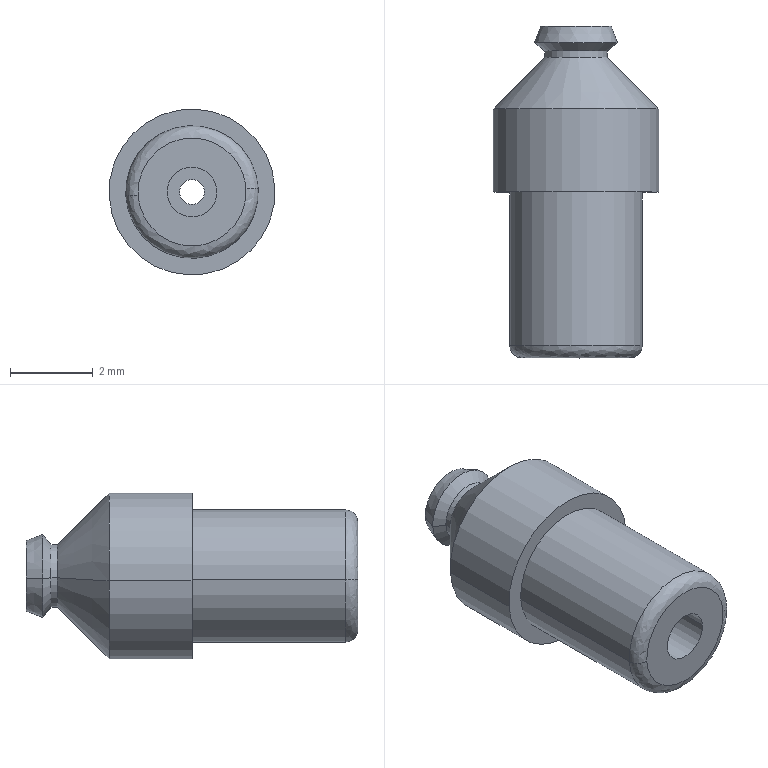Component | SolidWorks | HandlingMechanism-2_MVPTN2-3_2_2-1 | 1 solid | 23 faces | box 4 x 8 x 4 mm | volume 61 mm3 | cylinder 10 | cone 8 | plane 3 | spline 2 | commonest cylinder face diameters 3.2 x2 4 x2 1.2 x2 1.5 x2 0.6 x2
STEP:
#1=CARTESIAN_POINT('',(0.9678,9.134,9.249));
#2=VERTEX_POINT('',#1);
#3=CARTESIAN_POINT('',(1.07,9.134,9.255));
#4=VERTEX_POINT('',#3);
#5=CARTESIAN_POINT('',(0.9678,9.134,9.249));
#6=CARTESIAN_POINT('',(0.9617,9.134,9.351));
#7=CARTESIAN_POINT('',(1.064,9.134,9.357));
#8=CARTESIAN_POINT('',(1.07,9.134,9.255));
#9=(BOUNDED_CURVE()B_SPLINE_CURVE(3,(#5,#6,#7,#8),.UNSPECIFIED.,.F.,.F.)B_SPLINE_CURVE_WITH_KNOTS((4,4),(0.,1.),.UNSPECIFIED.)CURVE()GEOMETRIC_REPRESENTATION_ITEM()RATIONAL_B_SPLINE_CURVE((1.,0.3333,0.3333,1.))REPRESENTATION_ITEM(''));
#10=EDGE_CURVE('',#2,#4,#9,.T.);
#11=ORIENTED_EDGE('',*,*,#10,.T.);
#12=CARTESIAN_POINT('',(1.082,9.146,9.256));
#13=VERTEX_POINT('',#12);
#14=CARTESIAN_POINT('',(1.07,9.146,9.255));
#15=DIRECTION('',(-0.05953,-0.,0.9982));
#16=DIRECTION('',(0.9982,0.,0.05953));
#17=AXIS2_PLACEMENT_3D('',#14,#15,#16);
#18=CIRCLE('',#17,0.01181);
#19=EDGE_CURVE('',#4,#13,#18,.T.);
#20=ORIENTED_EDGE('',*,*,#19,.T.);
#21=CARTESIAN_POINT('',(0.956,9.146,9.248));
#22=VERTEX_POINT('',#21);
#23=CARTESIAN_POINT('',(1.019,9.146,9.252));
#24=DIRECTION('',(0.,1.,0.));
#25=DIRECTION('',(0.9982,0.,0.05953));
#26=AXIS2_PLACEMENT_3D('',#23,#24,#25);
#27=CIRCLE('',#26,0.06299);
#28=EDGE_CURVE('',#22,#13,#27,.T.);
#29=ORIENTED_EDGE('',*,*,#28,.F.);
#30=CARTESIAN_POINT('',(0.9678,9.146,9.249));
#31=DIRECTION('',(0.05953,0.,-0.9982));
#32=DIRECTION('',(-0.9982,0.,-0.05953));
#33=AXIS2_PLACEMENT_3D('',#30,#31,#32);
#34=CIRCLE('',#33,0.01181);
#35=EDGE_CURVE('',#2,#22,#34,.T.);
#36=ORIENTED_EDGE('',*,*,#35,.F.);
#37=EDGE_LOOP('',(#11,#20,#29,#36));
#38=FACE_OUTER_BOUND('',#37,.T.);
#39=CARTESIAN_POINT('',(1.07,9.134,9.255));
#40=CARTESIAN_POINT('',(1.064,9.134,9.357));
#41=CARTESIAN_POINT('',(0.9617,9.134,9.351));
#42=CARTESIAN_POINT('',(0.9678,9.134,9.249));
#43=CARTESIAN_POINT('',(1.077,9.134,9.255));
#44=CARTESIAN_POINT('',(1.07,9.134,9.371));
#45=CARTESIAN_POINT('',(0.954,9.134,9.365));
#46=CARTESIAN_POINT('',(0.9609,9.134,9.249));
#47=CARTESIAN_POINT('',(1.082,9.139,9.256));
#48=CARTESIAN_POINT('',(1.074,9.139,9.381));
#49=CARTESIAN_POINT('',(0.9485,9.139,9.374));
#50=CARTESIAN_POINT('',(0.956,9.139,9.248));
#51=CARTESIAN_POINT('',(1.082,9.146,9.256));
#52=CARTESIAN_POINT('',(1.074,9.146,9.381));
#53=CARTESIAN_POINT('',(0.9485,9.146,9.374));
#54=CARTESIAN_POINT('',(0.956,9.146,9.248));
#55=(BOUNDED_SURFACE()B_SPLINE_SURFACE(3,3,((#39,#40,#41,#42),(#43,#44,#45,#46),(#47,#48,#49,#50),(#51,#52,#53,#54)),.UNSPECIFIED.,.F.,.F.,.T.)B_SPLINE_SURFACE_WITH_KNOTS((4,4),(4,4),(0.,1.),(0.,1.),.UNSPECIFIED.)GEOMETRIC_REPRESENTATION_ITEM()RATIONAL_B_SPLINE_SURFACE(((1.,0.3333,0.3333,1.),(0.8047,0.2682,0.2682,0.8047),(0.8047,0.2682,0.2682,0.8047),(1.,0.3333,0.3333,1.)))REPRESENTATION_ITEM('')SURFACE());
#56=ADVANCED_FACE('',(#38),#55,.T.);
#57=CARTESIAN_POINT('',(1.019,9.146,9.252));
#58=DIRECTION('',(0.,1.,0.));
#59=DIRECTION('',(0.9982,0.,0.05953));
#60=AXIS2_PLACEMENT_3D('',#57,#58,#59);
#61=CIRCLE('',#60,0.06299);
#62=EDGE_CURVE('',#13,#22,#61,.T.);
#63=ORIENTED_EDGE('',*,*,#62,.T.);
#64=CARTESIAN_POINT('',(0.956,9.291,9.248));
#65=VERTEX_POINT('',#64);
#66=CARTESIAN_POINT('',(0.956,9.219,9.248));
#67=DIRECTION('',(0.,1.,0.));
#68=VECTOR('',#67,39.37);
#69=LINE('',#66,#68);
#70=EDGE_CURVE('',#22,#65,#69,.T.);
#71=ORIENTED_EDGE('',*,*,#70,.T.);
#72=CARTESIAN_POINT('',(1.082,9.291,9.256));
#73=VERTEX_POINT('',#72);
#74=CARTESIAN_POINT('',(1.019,9.291,9.252));
#75=DIRECTION('',(-0.,-1.,-0.));
#76=DIRECTION('',(0.9982,0.,0.05953));
#77=AXIS2_PLACEMENT_3D('',#74,#75,#76);
#78=CIRCLE('',#77,0.06299);
#79=EDGE_CURVE('',#65,#73,#78,.T.);
#80=ORIENTED_EDGE('',*,*,#79,.T.);
#81=CARTESIAN_POINT('',(1.082,9.219,9.256));
#82=DIRECTION('',(0.,1.,0.));
#83=VECTOR('',#82,39.37);
#84=LINE('',#81,#83);
#85=EDGE_CURVE('',#13,#73,#84,.T.);
#86=ORIENTED_EDGE('',*,*,#85,.F.);
#87=EDGE_LOOP('',(#63,#71,#80,#86));
#88=FACE_OUTER_BOUND('',#87,.T.);
#89=CARTESIAN_POINT('',(1.019,9.219,9.252));
#90=DIRECTION('',(0.,1.,0.));
#91=DIRECTION('',(0.9982,0.,0.05953));
#92=AXIS2_PLACEMENT_3D('',#89,#90,#91);
#93=CYLINDRICAL_SURFACE('',#92,0.06299);
#94=ADVANCED_FACE('',(#88),#93,.T.);
#95=CARTESIAN_POINT('',(0.9403,9.291,9.247));
#96=VERTEX_POINT('',#95);
#97=CARTESIAN_POINT('',(1.098,9.291,9.257));
#98=VERTEX_POINT('',#97);
#99=CARTESIAN_POINT('',(1.019,9.291,9.252));
#100=DIRECTION('',(-0.,-1.,-0.));
#101=DIRECTION('',(0.9982,0.,0.05953));
#102=AXIS2_PLACEMENT_3D('',#99,#100,#101);
#103=CIRCLE('',#102,0.07874);
#104=EDGE_CURVE('',#96,#98,#103,.T.);
#105=ORIENTED_EDGE('',*,*,#104,.F.);
#106=CARTESIAN_POINT('',(0.9403,9.37,9.247));
#107=VERTEX_POINT('',#106);
#108=CARTESIAN_POINT('',(0.9403,9.331,9.247));
#109=DIRECTION('',(0.,1.,0.));
#110=VECTOR('',#109,39.37);
#111=LINE('',#108,#110);
#112=EDGE_CURVE('',#96,#107,#111,.T.);
#113=ORIENTED_EDGE('',*,*,#112,.T.);
#114=CARTESIAN_POINT('',(1.098,9.37,9.257));
#115=VERTEX_POINT('',#114);
#116=CARTESIAN_POINT('',(1.019,9.37,9.252));
#117=DIRECTION('',(-0.,-1.,-0.));
#118=DIRECTION('',(0.9982,0.,0.05953));
#119=AXIS2_PLACEMENT_3D('',#116,#117,#118);
#120=CIRCLE('',#119,0.07874);
#121=EDGE_CURVE('',#107,#115,#120,.T.);
#122=ORIENTED_EDGE('',*,*,#121,.T.);
#123=CARTESIAN_POINT('',(1.098,9.331,9.257));
#124=DIRECTION('',(0.,1.,0.));
#125=VECTOR('',#124,39.37);
#126=LINE('',#123,#125);
#127=EDGE_CURVE('',#98,#115,#126,.T.);
#128=ORIENTED_EDGE('',*,*,#127,.F.);
#129=EDGE_LOOP('',(#105,#113,#122,#128));
#130=FACE_OUTER_BOUND('',#129,.T.);
#131=CARTESIAN_POINT('',(1.019,9.331,9.252));
#132=DIRECTION('',(0.,1.,0.));
#133=DIRECTION('',(0.9982,0.,0.05953));
#134=AXIS2_PLACEMENT_3D('',#131,#132,#133);
#135=CYLINDRICAL_SURFACE('',#134,0.07874);
#136=ADVANCED_FACE('',(#130),#135,.T.);
#137=CARTESIAN_POINT('',(0.9953,9.134,9.251));
#138=VERTEX_POINT('',#137);
#139=CARTESIAN_POINT('',(1.042,9.134,9.253));
#140=VERTEX_POINT('',#139);
#141=CARTESIAN_POINT('',(1.019,9.134,9.252));
#142=DIRECTION('',(0.,1.,0.));
#143=DIRECTION('',(0.9982,0.,0.05953));
#144=AXIS2_PLACEMENT_3D('',#141,#142,#143);
#145=CIRCLE('',#144,0.02362);
#146=EDGE_CURVE('',#138,#140,#145,.T.);
#147=ORIENTED_EDGE('',*,*,#146,.F.);
#148=CARTESIAN_POINT('',(0.9953,9.299,9.251));
#149=VERTEX_POINT('',#148);
#150=CARTESIAN_POINT('',(0.9953,9.217,9.251));
#151=DIRECTION('',(0.,1.,0.));
#152=VECTOR('',#151,39.37);
#153=LINE('',#150,#152);
#154=EDGE_CURVE('',#138,#149,#153,.T.);
#155=ORIENTED_EDGE('',*,*,#154,.T.);
#156=CARTESIAN_POINT('',(1.042,9.299,9.253));
#157=VERTEX_POINT('',#156);
#158=CARTESIAN_POINT('',(1.019,9.299,9.252));
#159=DIRECTION('',(-0.,-1.,-0.));
#160=DIRECTION('',(0.9982,0.,0.05953));
#161=AXIS2_PLACEMENT_3D('',#158,#159,#160);
#162=CIRCLE('',#161,0.02362);
#163=EDGE_CURVE('',#157,#149,#162,.T.);
#164=ORIENTED_EDGE('',*,*,#163,.F.);
#165=CARTESIAN_POINT('',(1.042,9.217,9.253));
#166=DIRECTION('',(0.,1.,0.));
#167=VECTOR('',#166,39.37);
#168=LINE('',#165,#167);
#169=EDGE_CURVE('',#140,#157,#168,.T.);
#170=ORIENTED_EDGE('',*,*,#169,.F.);
#171=EDGE_LOOP('',(#147,#155,#164,#170));
#172=FACE_OUTER_BOUND('',#171,.T.);
#173=CARTESIAN_POINT('',(1.019,9.217,9.252));
#174=DIRECTION('',(0.,1.,0.));
#175=DIRECTION('',(0.9982,0.,0.05953));
#176=AXIS2_PLACEMENT_3D('',#173,#174,#175);
#177=CYLINDRICAL_SURFACE('',#176,0.02362);
#178=ADVANCED_FACE('',(#172),#177,.F.);
#179=CARTESIAN_POINT('',(0.9894,9.419,9.25));
#180=VERTEX_POINT('',#179);
#181=CARTESIAN_POINT('',(1.048,9.419,9.254));
#182=VERTEX_POINT('',#181);
#183=CARTESIAN_POINT('',(1.019,9.419,9.252));
#184=DIRECTION('',(-0.,-1.,-0.));
#185=DIRECTION('',(0.05953,0.,-0.9982));
#186=AXIS2_PLACEMENT_3D('',#183,#184,#185);
#187=CIRCLE('',#186,0.02953);
#188=EDGE_CURVE('',#180,#182,#187,.T.);
#189=ORIENTED_EDGE('',*,*,#188,.T.);
#190=CARTESIAN_POINT('',(1.098,9.37,9.257));
#191=DIRECTION('',(0.7059,-0.7071,0.04209));
#192=VECTOR('',#191,39.37);
#193=LINE('',#190,#192);
#194=EDGE_CURVE('',#182,#115,#193,.T.);
#195=ORIENTED_EDGE('',*,*,#194,.T.);
#196=ORIENTED_EDGE('',*,*,#121,.F.);
#197=CARTESIAN_POINT('',(0.9403,9.37,9.247));
#198=DIRECTION('',(-0.7059,-0.7071,-0.04209));
#199=VECTOR('',#198,39.37);
#200=LINE('',#197,#199);
#201=EDGE_CURVE('',#180,#107,#200,.T.);
#202=ORIENTED_EDGE('',*,*,#201,.F.);
#203=EDGE_LOOP('',(#189,#195,#196,#202));
#204=FACE_OUTER_BOUND('',#203,.T.);
#205=CARTESIAN_POINT('',(1.019,9.37,9.252));
#206=DIRECTION('',(-0.,-1.,-0.));
#207=DIRECTION('',(-0.9982,0.,-0.05953));
#208=AXIS2_PLACEMENT_3D('',#205,#206,#207);
#209=CONICAL_SURFACE('',#208,0.07874,0.7854);
#210=ADVANCED_FACE('',(#204),#209,.T.);
#211=ORIENTED_EDGE('',*,*,#188,.F.);
#212=CARTESIAN_POINT('',(0.9894,9.425,9.25));
#213=VERTEX_POINT('',#212);
#214=CARTESIAN_POINT('',(0.9894,9.422,9.25));
#215=DIRECTION('',(0.,1.,0.));
#216=VECTOR('',#215,39.37);
#217=LINE('',#214,#216);
#218=EDGE_CURVE('',#180,#213,#217,.T.);
#219=ORIENTED_EDGE('',*,*,#218,.T.);
#220=CARTESIAN_POINT('',(1.048,9.425,9.254));
#221=VERTEX_POINT('',#220);
#222=CARTESIAN_POINT('',(1.019,9.425,9.252));
#223=DIRECTION('',(-0.,-1.,-0.));
#224=DIRECTION('',(0.9982,0.,0.05953));
#225=AXIS2_PLACEMENT_3D('',#222,#223,#224);
#226=CIRCLE('',#225,0.02953);
#227=EDGE_CURVE('',#213,#221,#226,.T.);
#228=ORIENTED_EDGE('',*,*,#227,.T.);
#229=CARTESIAN_POINT('',(1.048,9.422,9.254));
#230=DIRECTION('',(0.,1.,0.));
#231=VECTOR('',#230,39.37);
#232=LINE('',#229,#231);
#233=EDGE_CURVE('',#182,#221,#232,.T.);
#234=ORIENTED_EDGE('',*,*,#233,.F.);
#235=EDGE_LOOP('',(#211,#219,#228,#234));
#236=FACE_OUTER_BOUND('',#235,.T.);
#237=CARTESIAN_POINT('',(1.019,9.422,9.252));
#238=DIRECTION('',(0.,1.,0.));
#239=DIRECTION('',(0.9982,0.,0.05953));
#240=AXIS2_PLACEMENT_3D('',#237,#238,#239);
#241=CYLINDRICAL_SURFACE('',#240,0.02953);
#242=ADVANCED_FACE('',(#236),#241,.T.);
#243=CARTESIAN_POINT('',(1.031,9.299,9.253));
#244=VERTEX_POINT('',#243);
#245=CARTESIAN_POINT('',(1.007,9.299,9.251));
#246=VERTEX_POINT('',#245);
#247=CARTESIAN_POINT('',(1.019,9.299,9.252));
#248=DIRECTION('',(-0.,-1.,-0.));
#249=DIRECTION('',(0.9982,0.,0.05953));
#250=AXIS2_PLACEMENT_3D('',#247,#248,#249);
#251=CIRCLE('',#250,0.01181);
#252=EDGE_CURVE('',#244,#246,#251,.T.);
#253=ORIENTED_EDGE('',*,*,#252,.T.);
#254=CARTESIAN_POINT('',(1.007,9.441,9.251));
#255=VERTEX_POINT('',#254);
#256=CARTESIAN_POINT('',(1.007,9.37,9.251));
#257=DIRECTION('',(0.,1.,0.));
#258=VECTOR('',#257,39.37);
#259=LINE('',#256,#258);
#260=EDGE_CURVE('',#246,#255,#259,.T.);
#261=ORIENTED_EDGE('',*,*,#260,.T.);
#262=CARTESIAN_POINT('',(1.031,9.441,9.253));
#263=VERTEX_POINT('',#262);
#264=CARTESIAN_POINT('',(1.019,9.441,9.252));
#265=DIRECTION('',(-0.,-1.,-0.));
#266=DIRECTION('',(0.9982,0.,0.05953));
#267=AXIS2_PLACEMENT_3D('',#264,#265,#266);
#268=CIRCLE('',#267,0.01181);
#269=EDGE_CURVE('',#263,#255,#268,.T.);
#270=ORIENTED_EDGE('',*,*,#269,.F.);
#271=CARTESIAN_POINT('',(1.031,9.37,9.253));
#272=DIRECTION('',(0.,1.,0.));
#273=VECTOR('',#272,39.37);
#274=LINE('',#271,#273);
#275=EDGE_CURVE('',#244,#263,#274,.T.);
#276=ORIENTED_EDGE('',*,*,#275,.F.);
#277=EDGE_LOOP('',(#253,#261,#270,#276));
#278=FACE_OUTER_BOUND('',#277,.T.);
#279=CARTESIAN_POINT('',(1.019,9.37,9.252));
#280=DIRECTION('',(0.,1.,0.));
#281=DIRECTION('',(0.9982,0.,0.05953));
#282=AXIS2_PLACEMENT_3D('',#279,#280,#281);
#283=CYLINDRICAL_SURFACE('',#282,0.01181);
#284=ADVANCED_FACE('',(#278),#283,.F.);
#285=ORIENTED_EDGE('',*,*,#227,.F.);
#286=CARTESIAN_POINT('',(0.9796,9.433,9.25));
#287=VERTEX_POINT('',#286);
#288=CARTESIAN_POINT('',(0.9796,9.433,9.25));
#289=DIRECTION('',(-0.7795,0.6247,-0.04648));
#290=VECTOR('',#289,39.37);
#291=LINE('',#288,#290);
#292=EDGE_CURVE('',#213,#287,#291,.T.);
#293=ORIENTED_EDGE('',*,*,#292,.T.);
#294=CARTESIAN_POINT('',(1.058,9.433,9.254));
#295=VERTEX_POINT('',#294);
#296=CARTESIAN_POINT('',(1.019,9.433,9.252));
#297=DIRECTION('',(-0.,-1.,-0.));
#298=DIRECTION('',(0.05953,0.,-0.9982));
#299=AXIS2_PLACEMENT_3D('',#296,#297,#298);
#300=CIRCLE('',#299,0.03937);
#301=EDGE_CURVE('',#287,#295,#300,.T.);
#302=ORIENTED_EDGE('',*,*,#301,.T.);
#303=CARTESIAN_POINT('',(1.058,9.433,9.254));
#304=DIRECTION('',(0.7795,0.6247,0.04648));
#305=VECTOR('',#304,39.37);
#306=LINE('',#303,#305);
#307=EDGE_CURVE('',#221,#295,#306,.T.);
#308=ORIENTED_EDGE('',*,*,#307,.F.);
#309=EDGE_LOOP('',(#285,#293,#302,#308));
#310=FACE_OUTER_BOUND('',#309,.T.);
#311=CARTESIAN_POINT('',(1.019,9.433,9.252));
#312=DIRECTION('',(0.,1.,0.));
#313=DIRECTION('',(0.9982,0.,0.05953));
#314=AXIS2_PLACEMENT_3D('',#311,#312,#313);
#315=CONICAL_SURFACE('',#314,0.03937,0.8961);
#316=ADVANCED_FACE('',(#310),#315,.T.);
#317=ORIENTED_EDGE('',*,*,#269,.T.);
#318=CARTESIAN_POINT('',(0.9855,9.449,9.25));
#319=VERTEX_POINT('',#318);
#320=CARTESIAN_POINT('',(0.9855,9.449,9.25));
#321=DIRECTION('',(-0.9381,0.3417,-0.05594));
#322=VECTOR('',#321,39.37);
#323=LINE('',#320,#322);
#324=EDGE_CURVE('',#255,#319,#323,.T.);
#325=ORIENTED_EDGE('',*,*,#324,.T.);
#326=CARTESIAN_POINT('',(1.052,9.449,9.254));
#327=VERTEX_POINT('',#326);
#328=CARTESIAN_POINT('',(1.019,9.449,9.252));
#329=DIRECTION('',(-0.,-1.,-0.));
#330=DIRECTION('',(0.05953,0.,-0.9982));
#331=AXIS2_PLACEMENT_3D('',#328,#329,#330);
#332=CIRCLE('',#331,0.03346);
#333=EDGE_CURVE('',#327,#319,#332,.T.);
#334=ORIENTED_EDGE('',*,*,#333,.F.);
#335=CARTESIAN_POINT('',(1.052,9.449,9.254));
#336=DIRECTION('',(0.9381,0.3417,0.05594));
#337=VECTOR('',#336,39.37);
#338=LINE('',#335,#337);
#339=EDGE_CURVE('',#263,#327,#338,.T.);
#340=ORIENTED_EDGE('',*,*,#339,.F.);
#341=EDGE_LOOP('',(#317,#325,#334,#340));
#342=FACE_OUTER_BOUND('',#341,.T.);
#343=CARTESIAN_POINT('',(1.019,9.449,9.252));
#344=DIRECTION('',(0.,1.,0.));
#345=DIRECTION('',(0.9982,0.,0.05953));
#346=AXIS2_PLACEMENT_3D('',#343,#344,#345);
#347=CONICAL_SURFACE('',#346,0.03346,1.222);
#348=ADVANCED_FACE('',(#342),#347,.F.);
#349=CARTESIAN_POINT('',(1.019,9.449,9.252));
#350=DIRECTION('',(-0.,-1.,-0.));
#351=DIRECTION('',(0.05953,0.,-0.9982));
#352=AXIS2_PLACEMENT_3D('',#349,#350,#351);
#353=CIRCLE('',#352,0.03346);
#354=EDGE_CURVE('',#319,#327,#353,.T.);
#355=ORIENTED_EDGE('',*,*,#354,.T.);
#356=CARTESIAN_POINT('',(1.058,9.433,9.254));
#357=DIRECTION('',(0.3505,-0.9363,0.0209));
#358=VECTOR('',#357,39.37);
#359=LINE('',#356,#358);
#360=EDGE_CURVE('',#327,#295,#359,.T.);
#361=ORIENTED_EDGE('',*,*,#360,.T.);
#362=ORIENTED_EDGE('',*,*,#301,.F.);
#363=CARTESIAN_POINT('',(0.9796,9.433,9.25));
#364=DIRECTION('',(-0.3505,-0.9363,-0.0209));
#365=VECTOR('',#364,39.37);
#366=LINE('',#363,#365);
#367=EDGE_CURVE('',#319,#287,#366,.T.);
#368=ORIENTED_EDGE('',*,*,#367,.F.);
#369=EDGE_LOOP('',(#355,#361,#362,#368));
#370=FACE_OUTER_BOUND('',#369,.T.);
#371=CARTESIAN_POINT('',(1.019,9.433,9.252));
#372=DIRECTION('',(-0.,-1.,-0.));
#373=DIRECTION('',(-0.9982,0.,-0.05953));
#374=AXIS2_PLACEMENT_3D('',#371,#372,#373);
#375=CONICAL_SURFACE('',#374,0.03937,0.3588);
#376=ADVANCED_FACE('',(#370),#375,.T.);
#377=ORIENTED_EDGE('',*,*,#70,.F.);
#378=ORIENTED_EDGE('',*,*,#28,.T.);
#379=ORIENTED_EDGE('',*,*,#85,.T.);
#380=CARTESIAN_POINT('',(1.019,9.291,9.252));
#381=DIRECTION('',(-0.,-1.,-0.));
#382=DIRECTION('',(0.9982,0.,0.05953));
#383=AXIS2_PLACEMENT_3D('',#380,#381,#382);
#384=CIRCLE('',#383,0.06299);
#385=EDGE_CURVE('',#73,#65,#384,.T.);
#386=ORIENTED_EDGE('',*,*,#385,.T.);
#387=EDGE_LOOP('',(#377,#378,#379,#386));
#388=FACE_OUTER_BOUND('',#387,.T.);
#389=CARTESIAN_POINT('',(1.019,9.219,9.252));
#390=DIRECTION('',(0.,1.,0.));
#391=DIRECTION('',(0.9982,0.,0.05953));
#392=AXIS2_PLACEMENT_3D('',#389,#390,#391);
#393=CYLINDRICAL_SURFACE('',#392,0.06299);
#394=ADVANCED_FACE('',(#388),#393,.T.);
#395=ORIENTED_EDGE('',*,*,#19,.F.);
#396=CARTESIAN_POINT('',(1.022,9.134,9.201));
#397=VERTEX_POINT('',#396);
#398=CARTESIAN_POINT('',(1.07,9.134,9.255));
#399=CARTESIAN_POINT('',(1.072,9.134,9.225));
#400=CARTESIAN_POINT('',(1.052,9.134,9.203));
#401=CARTESIAN_POINT('',(1.022,9.134,9.201));
#402=(BOUNDED_CURVE()B_SPLINE_CURVE(3,(#398,#399,#400,#401),.UNSPECIFIED.,.F.,.T.)B_SPLINE_CURVE_WITH_KNOTS((4,4),(0.,1.),.UNSPECIFIED.)CURVE()GEOMETRIC_REPRESENTATION_ITEM()RATIONAL_B_SPLINE_CURVE((1.,0.8047,0.8047,1.))REPRESENTATION_ITEM(''));
#403=EDGE_CURVE('',#4,#397,#402,.T.);
#404=ORIENTED_EDGE('',*,*,#403,.T.);
#405=CARTESIAN_POINT('',(1.022,9.134,9.201));
#406=CARTESIAN_POINT('',(0.992,9.134,9.199));
#407=CARTESIAN_POINT('',(0.9696,9.134,9.219));
#408=CARTESIAN_POINT('',(0.9678,9.134,9.249));
#409=(BOUNDED_CURVE()B_SPLINE_CURVE(3,(#405,#406,#407,#408),.UNSPECIFIED.,.F.,.F.)B_SPLINE_CURVE_WITH_KNOTS((4,4),(0.,1.),.UNSPECIFIED.)CURVE()GEOMETRIC_REPRESENTATION_ITEM()RATIONAL_B_SPLINE_CURVE((1.,0.8047,0.8047,1.))REPRESENTATION_ITEM(''));
#410=EDGE_CURVE('',#397,#2,#409,.T.);
#411=ORIENTED_EDGE('',*,*,#410,.T.);
#412=ORIENTED_EDGE('',*,*,#35,.T.);
#413=ORIENTED_EDGE('',*,*,#62,.F.);
#414=EDGE_LOOP('',(#395,#404,#411,#412,#413));
#415=FACE_OUTER_BOUND('',#414,.T.);
#416=CARTESIAN_POINT('',(0.9678,9.134,9.249));
#417=CARTESIAN_POINT('',(0.9739,9.134,9.147));
#418=CARTESIAN_POINT('',(1.076,9.134,9.153));
#419=CARTESIAN_POINT('',(1.07,9.134,9.255));
#420=CARTESIAN_POINT('',(0.9609,9.134,9.249));
#421=CARTESIAN_POINT('',(0.9678,9.134,9.133));
#422=CARTESIAN_POINT('',(1.084,9.134,9.139));
#423=CARTESIAN_POINT('',(1.077,9.134,9.255));
#424=CARTESIAN_POINT('',(0.956,9.139,9.248));
#425=CARTESIAN_POINT('',(0.9635,9.139,9.122));
#426=CARTESIAN_POINT('',(1.089,9.139,9.13));
#427=CARTESIAN_POINT('',(1.082,9.139,9.256));
#428=CARTESIAN_POINT('',(0.956,9.146,9.248));
#429=CARTESIAN_POINT('',(0.9635,9.146,9.122));
#430=CARTESIAN_POINT('',(1.089,9.146,9.13));
#431=CARTESIAN_POINT('',(1.082,9.146,9.256));
#432=(BOUNDED_SURFACE()B_SPLINE_SURFACE(3,3,((#416,#417,#418,#419),(#420,#421,#422,#423),(#424,#425,#426,#427),(#428,#429,#430,#431)),.UNSPECIFIED.,.F.,.F.,.T.)B_SPLINE_SURFACE_WITH_KNOTS((4,4),(4,4),(0.,1.),(0.,1.),.UNSPECIFIED.)GEOMETRIC_REPRESENTATION_ITEM()RATIONAL_B_SPLINE_SURFACE(((1.,0.3333,0.3333,1.),(0.8047,0.2682,0.2682,0.8047),(0.8047,0.2682,0.2682,0.8047),(1.,0.3333,0.3333,1.)))REPRESENTATION_ITEM('')SURFACE());
#433=ADVANCED_FACE('',(#415),#432,.T.);
#434=CARTESIAN_POINT('',(1.019,9.291,9.252));
#435=DIRECTION('',(-0.,-1.,-0.));
#436=DIRECTION('',(0.9982,0.,0.05953));
#437=AXIS2_PLACEMENT_3D('',#434,#435,#436);
#438=CIRCLE('',#437,0.07874);
#439=EDGE_CURVE('',#98,#96,#438,.T.);
#440=ORIENTED_EDGE('',*,*,#439,.T.);
#441=ORIENTED_EDGE('',*,*,#104,.T.);
#442=EDGE_LOOP('',(#440,#441));
#443=FACE_OUTER_BOUND('',#442,.T.);
#444=ORIENTED_EDGE('',*,*,#385,.F.);
#445=ORIENTED_EDGE('',*,*,#79,.F.);
#446=EDGE_LOOP('',(#444,#445));
#447=FACE_BOUND('',#446,.T.);
#448=CARTESIAN_POINT('',(1.023,9.291,9.181));
#449=DIRECTION('',(-0.,-1.,-0.));
#450=DIRECTION('',(-0.9982,0.,-0.05953));
#451=AXIS2_PLACEMENT_3D('',#448,#449,#450);
#452=PLANE('',#451);
#453=ADVANCED_FACE('',(#443,#447),#452,.T.);
#454=ORIENTED_EDGE('',*,*,#10,.F.);
#455=ORIENTED_EDGE('',*,*,#410,.F.);
#456=ORIENTED_EDGE('',*,*,#403,.F.);
#457=EDGE_LOOP('',(#454,#455,#456));
#458=FACE_OUTER_BOUND('',#457,.T.);
#459=CARTESIAN_POINT('',(1.019,9.134,9.252));
#460=DIRECTION('',(0.,1.,0.));
#461=DIRECTION('',(0.9982,0.,0.05953));
#462=AXIS2_PLACEMENT_3D('',#459,#460,#461);
#463=CIRCLE('',#462,0.02362);
#464=EDGE_CURVE('',#140,#138,#463,.T.);
#465=ORIENTED_EDGE('',*,*,#464,.T.);
#466=ORIENTED_EDGE('',*,*,#146,.T.);
#467=EDGE_LOOP('',(#465,#466));
#468=FACE_BOUND('',#467,.T.);
#469=CARTESIAN_POINT('',(1.02,9.134,9.226));
#470=DIRECTION('',(-0.,-1.,-0.));
#471=DIRECTION('',(-0.9982,0.,-0.05953));
#472=AXIS2_PLACEMENT_3D('',#469,#470,#471);
#473=PLANE('',#472);
#474=ADVANCED_FACE('',(#458,#468),#473,.T.);
#475=ORIENTED_EDGE('',*,*,#112,.F.);
#476=ORIENTED_EDGE('',*,*,#439,.F.);
#477=ORIENTED_EDGE('',*,*,#127,.T.);
#478=CARTESIAN_POINT('',(1.019,9.37,9.252));
#479=DIRECTION('',(-0.,-1.,-0.));
#480=DIRECTION('',(0.9982,0.,0.05953));
#481=AXIS2_PLACEMENT_3D('',#478,#479,#480);
#482=CIRCLE('',#481,0.07874);
#483=EDGE_CURVE('',#115,#107,#482,.T.);
#484=ORIENTED_EDGE('',*,*,#483,.T.);
#485=EDGE_LOOP('',(#475,#476,#477,#484));
#486=FACE_OUTER_BOUND('',#485,.T.);
#487=CARTESIAN_POINT('',(1.019,9.331,9.252));
#488=DIRECTION('',(0.,1.,0.));
#489=DIRECTION('',(0.9982,0.,0.05953));
#490=AXIS2_PLACEMENT_3D('',#487,#488,#489);
#491=CYLINDRICAL_SURFACE('',#490,0.07874);
#492=ADVANCED_FACE('',(#486),#491,.T.);
#493=ORIENTED_EDGE('',*,*,#154,.F.);
#494=ORIENTED_EDGE('',*,*,#464,.F.);
#495=ORIENTED_EDGE('',*,*,#169,.T.);
#496=CARTESIAN_POINT('',(1.019,9.299,9.252));
#497=DIRECTION('',(-0.,-1.,-0.));
#498=DIRECTION('',(0.9982,0.,0.05953));
#499=AXIS2_PLACEMENT_3D('',#496,#497,#498);
#500=CIRCLE('',#499,0.02362);
#501=EDGE_CURVE('',#149,#157,#500,.T.);
#502=ORIENTED_EDGE('',*,*,#501,.F.);
#503=EDGE_LOOP('',(#493,#494,#495,#502));
#504=FACE_OUTER_BOUND('',#503,.T.);
#505=CARTESIAN_POINT('',(1.019,9.217,9.252));
#506=DIRECTION('',(0.,1.,0.));
#507=DIRECTION('',(0.9982,0.,0.05953));
#508=AXIS2_PLACEMENT_3D('',#505,#506,#507);
#509=CYLINDRICAL_SURFACE('',#508,0.02362);
#510=ADVANCED_FACE('',(#504),#509,.F.);
#511=ORIENTED_EDGE('',*,*,#194,.F.);
#512=CARTESIAN_POINT('',(1.019,9.419,9.252));
#513=DIRECTION('',(-0.,-1.,-0.));
#514=DIRECTION('',(0.05953,0.,-0.9982));
#515=AXIS2_PLACEMENT_3D('',#512,#513,#514);
#516=CIRCLE('',#515,0.02953);
#517=EDGE_CURVE('',#182,#180,#516,.T.);
#518=ORIENTED_EDGE('',*,*,#517,.T.);
#519=ORIENTED_EDGE('',*,*,#201,.T.);
#520=ORIENTED_EDGE('',*,*,#483,.F.);
#521=EDGE_LOOP('',(#511,#518,#519,#520));
#522=FACE_OUTER_BOUND('',#521,.T.);
#523=CARTESIAN_POINT('',(1.019,9.37,9.252));
#524=DIRECTION('',(-0.,-1.,-0.));
#525=DIRECTION('',(-0.9982,0.,-0.05953));
#526=AXIS2_PLACEMENT_3D('',#523,#524,#525);
#527=CONICAL_SURFACE('',#526,0.07874,0.7854);
#528=ADVANCED_FACE('',(#522),#527,.T.);
#529=ORIENTED_EDGE('',*,*,#252,.F.);
#530=CARTESIAN_POINT('',(1.019,9.299,9.252));
#531=DIRECTION('',(-0.,-1.,-0.));
#532=DIRECTION('',(0.9982,0.,0.05953));
#533=AXIS2_PLACEMENT_3D('',#530,#531,#532);
#534=CIRCLE('',#533,0.01181);
#535=EDGE_CURVE('',#246,#244,#534,.T.);
#536=ORIENTED_EDGE('',*,*,#535,.F.);
#537=EDGE_LOOP('',(#529,#536));
#538=FACE_BOUND('',#537,.T.);
#539=ORIENTED_EDGE('',*,*,#163,.T.);
#540=ORIENTED_EDGE('',*,*,#501,.T.);
#541=EDGE_LOOP('',(#539,#540));
#542=FACE_OUTER_BOUND('',#541,.T.);
#543=CARTESIAN_POINT('',(1.02,9.299,9.234));
#544=DIRECTION('',(0.,1.,0.));
#545=DIRECTION('',(0.9982,-0.,0.05953));
#546=AXIS2_PLACEMENT_3D('',#543,#544,#545);
#547=PLANE('',#546);
#548=ADVANCED_FACE('',(#538,#542),#547,.F.);
#549=ORIENTED_EDGE('',*,*,#218,.F.);
#550=ORIENTED_EDGE('',*,*,#517,.F.);
#551=ORIENTED_EDGE('',*,*,#233,.T.);
#552=CARTESIAN_POINT('',(1.019,9.425,9.252));
#553=DIRECTION('',(-0.,-1.,-0.));
#554=DIRECTION('',(0.9982,0.,0.05953));
#555=AXIS2_PLACEMENT_3D('',#552,#553,#554);
#556=CIRCLE('',#555,0.02953);
#557=EDGE_CURVE('',#221,#213,#556,.T.);
#558=ORIENTED_EDGE('',*,*,#557,.T.);
#559=EDGE_LOOP('',(#549,#550,#551,#558));
#560=FACE_OUTER_BOUND('',#559,.T.);
#561=CARTESIAN_POINT('',(1.019,9.422,9.252));
#562=DIRECTION('',(0.,1.,0.));
#563=DIRECTION('',(0.9982,0.,0.05953));
#564=AXIS2_PLACEMENT_3D('',#561,#562,#563);
#565=CYLINDRICAL_SURFACE('',#564,0.02953);
#566=ADVANCED_FACE('',(#560),#565,.T.);
#567=ORIENTED_EDGE('',*,*,#260,.F.);
#568=ORIENTED_EDGE('',*,*,#535,.T.);
#569=ORIENTED_EDGE('',*,*,#275,.T.);
#570=CARTESIAN_POINT('',(1.019,9.441,9.252));
#571=DIRECTION('',(-0.,-1.,-0.));
#572=DIRECTION('',(0.9982,0.,0.05953));
#573=AXIS2_PLACEMENT_3D('',#570,#571,#572);
#574=CIRCLE('',#573,0.01181);
#575=EDGE_CURVE('',#255,#263,#574,.T.);
#576=ORIENTED_EDGE('',*,*,#575,.F.);
#577=EDGE_LOOP('',(#567,#568,#569,#576));
#578=FACE_OUTER_BOUND('',#577,.T.);
#579=CARTESIAN_POINT('',(1.019,9.37,9.252));
#580=DIRECTION('',(0.,1.,0.));
#581=DIRECTION('',(0.9982,0.,0.05953));
#582=AXIS2_PLACEMENT_3D('',#579,#580,#581);
#583=CYLINDRICAL_SURFACE('',#582,0.01181);
#584=ADVANCED_FACE('',(#578),#583,.F.);
#585=ORIENTED_EDGE('',*,*,#292,.F.);
#586=ORIENTED_EDGE('',*,*,#557,.F.);
#587=ORIENTED_EDGE('',*,*,#307,.T.);
#588=CARTESIAN_POINT('',(1.019,9.433,9.252));
#589=DIRECTION('',(-0.,-1.,-0.));
#590=DIRECTION('',(0.05953,0.,-0.9982));
#591=AXIS2_PLACEMENT_3D('',#588,#589,#590);
#592=CIRCLE('',#591,0.03937);
#593=EDGE_CURVE('',#295,#287,#592,.T.);
#594=ORIENTED_EDGE('',*,*,#593,.T.);
#595=EDGE_LOOP('',(#585,#586,#587,#594));
#596=FACE_OUTER_BOUND('',#595,.T.);
#597=CARTESIAN_POINT('',(1.019,9.433,9.252));
#598=DIRECTION('',(0.,1.,0.));
#599=DIRECTION('',(0.9982,0.,0.05953));
#600=AXIS2_PLACEMENT_3D('',#597,#598,#599);
#601=CONICAL_SURFACE('',#600,0.03937,0.8961);
#602=ADVANCED_FACE('',(#596),#601,.T.);
#603=ORIENTED_EDGE('',*,*,#324,.F.);
#604=ORIENTED_EDGE('',*,*,#575,.T.);
#605=ORIENTED_EDGE('',*,*,#339,.T.);
#606=ORIENTED_EDGE('',*,*,#354,.F.);
#607=EDGE_LOOP('',(#603,#604,#605,#606));
#608=FACE_OUTER_BOUND('',#607,.T.);
#609=CARTESIAN_POINT('',(1.019,9.449,9.252));
#610=DIRECTION('',(0.,1.,0.));
#611=DIRECTION('',(0.9982,0.,0.05953));
#612=AXIS2_PLACEMENT_3D('',#609,#610,#611);
#613=CONICAL_SURFACE('',#612,0.03346,1.222);
#614=ADVANCED_FACE('',(#608),#613,.F.);
#615=ORIENTED_EDGE('',*,*,#360,.F.);
#616=ORIENTED_EDGE('',*,*,#333,.T.);
#617=ORIENTED_EDGE('',*,*,#367,.T.);
#618=ORIENTED_EDGE('',*,*,#593,.F.);
#619=EDGE_LOOP('',(#615,#616,#617,#618));
#620=FACE_OUTER_BOUND('',#619,.T.);
#621=CARTESIAN_POINT('',(1.019,9.433,9.252));
#622=DIRECTION('',(-0.,-1.,-0.));
#623=DIRECTION('',(-0.9982,0.,-0.05953));
#624=AXIS2_PLACEMENT_3D('',#621,#622,#623);
#625=CONICAL_SURFACE('',#624,0.03937,0.3588);
#626=ADVANCED_FACE('',(#620),#625,.T.);
#627=CLOSED_SHELL('',(#56,#94,#136,#178,#210,#242,#284,#316,#348,#376,#394,#433,#453,#474,#492,#510,#528,#548,#566,#584,#602,#614,#626));
#628=MANIFOLD_SOLID_BREP('',#627);
#629=CARTESIAN_POINT('',(0.,0.,0.));
#630=DIRECTION('',(0.,0.,1.));
#631=DIRECTION('',(1.,0.,0.));
#632=AXIS2_PLACEMENT_3D('',#629,#630,#631);
#633=(LENGTH_UNIT()NAMED_UNIT(*)SI_UNIT($,.METRE.));
#634=LENGTH_MEASURE_WITH_UNIT(LENGTH_MEASURE(0.0254),#633);
#635=DIMENSIONAL_EXPONENTS(1.,0.,0.,0.,0.,0.,0.);
#636=(CONVERSION_BASED_UNIT('',#634)LENGTH_UNIT()NAMED_UNIT(#635));
#637=UNCERTAINTY_MEASURE_WITH_UNIT(LENGTH_MEASURE(0.00001),#636,'','');
#638=(NAMED_UNIT(*)PLANE_ANGLE_UNIT()SI_UNIT($,.RADIAN.));
#639=(NAMED_UNIT(*)SI_UNIT($,.STERADIAN.)SOLID_ANGLE_UNIT());
#640=(GEOMETRIC_REPRESENTATION_CONTEXT(3)GLOBAL_UNCERTAINTY_ASSIGNED_CONTEXT((#637))GLOBAL_UNIT_ASSIGNED_CONTEXT((#636,#638,#639))REPRESENTATION_CONTEXT('',''));
#641=ADVANCED_BREP_SHAPE_REPRESENTATION('',(#628,#632),#640);
#642=COLOUR_RGB('',0.7922,0.8196,0.9333);
#643=FILL_AREA_STYLE_COLOUR('',#642);
#644=FILL_AREA_STYLE('',(#643));
#645=SURFACE_STYLE_FILL_AREA(#644);
#646=SURFACE_SIDE_STYLE('',(#645));
#647=SURFACE_STYLE_USAGE(.BOTH.,#646);
#648=PRESENTATION_STYLE_ASSIGNMENT((#647));
#649=STYLED_ITEM('',(#648),#628);
#650=PRESENTATION_LAYER_ASSIGNMENT('','',(#649));
#651=(LENGTH_UNIT()NAMED_UNIT(*)SI_UNIT($,.METRE.));
#652=LENGTH_MEASURE_WITH_UNIT(LENGTH_MEASURE(0.0254),#651);
#653=DIMENSIONAL_EXPONENTS(1.,0.,0.,0.,0.,0.,0.);
#654=(CONVERSION_BASED_UNIT('',#652)LENGTH_UNIT()NAMED_UNIT(#653));
#655=UNCERTAINTY_MEASURE_WITH_UNIT(LENGTH_MEASURE(0.00001),#654,'','');
#656=(NAMED_UNIT(*)PLANE_ANGLE_UNIT()SI_UNIT($,.RADIAN.));
#657=(NAMED_UNIT(*)SI_UNIT($,.STERADIAN.)SOLID_ANGLE_UNIT());
#658=(GEOMETRIC_REPRESENTATION_CONTEXT(3)GLOBAL_UNCERTAINTY_ASSIGNED_CONTEXT((#655))GLOBAL_UNIT_ASSIGNED_CONTEXT((#654,#656,#657))REPRESENTATION_CONTEXT('',''));
#659=MECHANICAL_DESIGN_GEOMETRIC_PRESENTATION_REPRESENTATION('',(#649),#658);